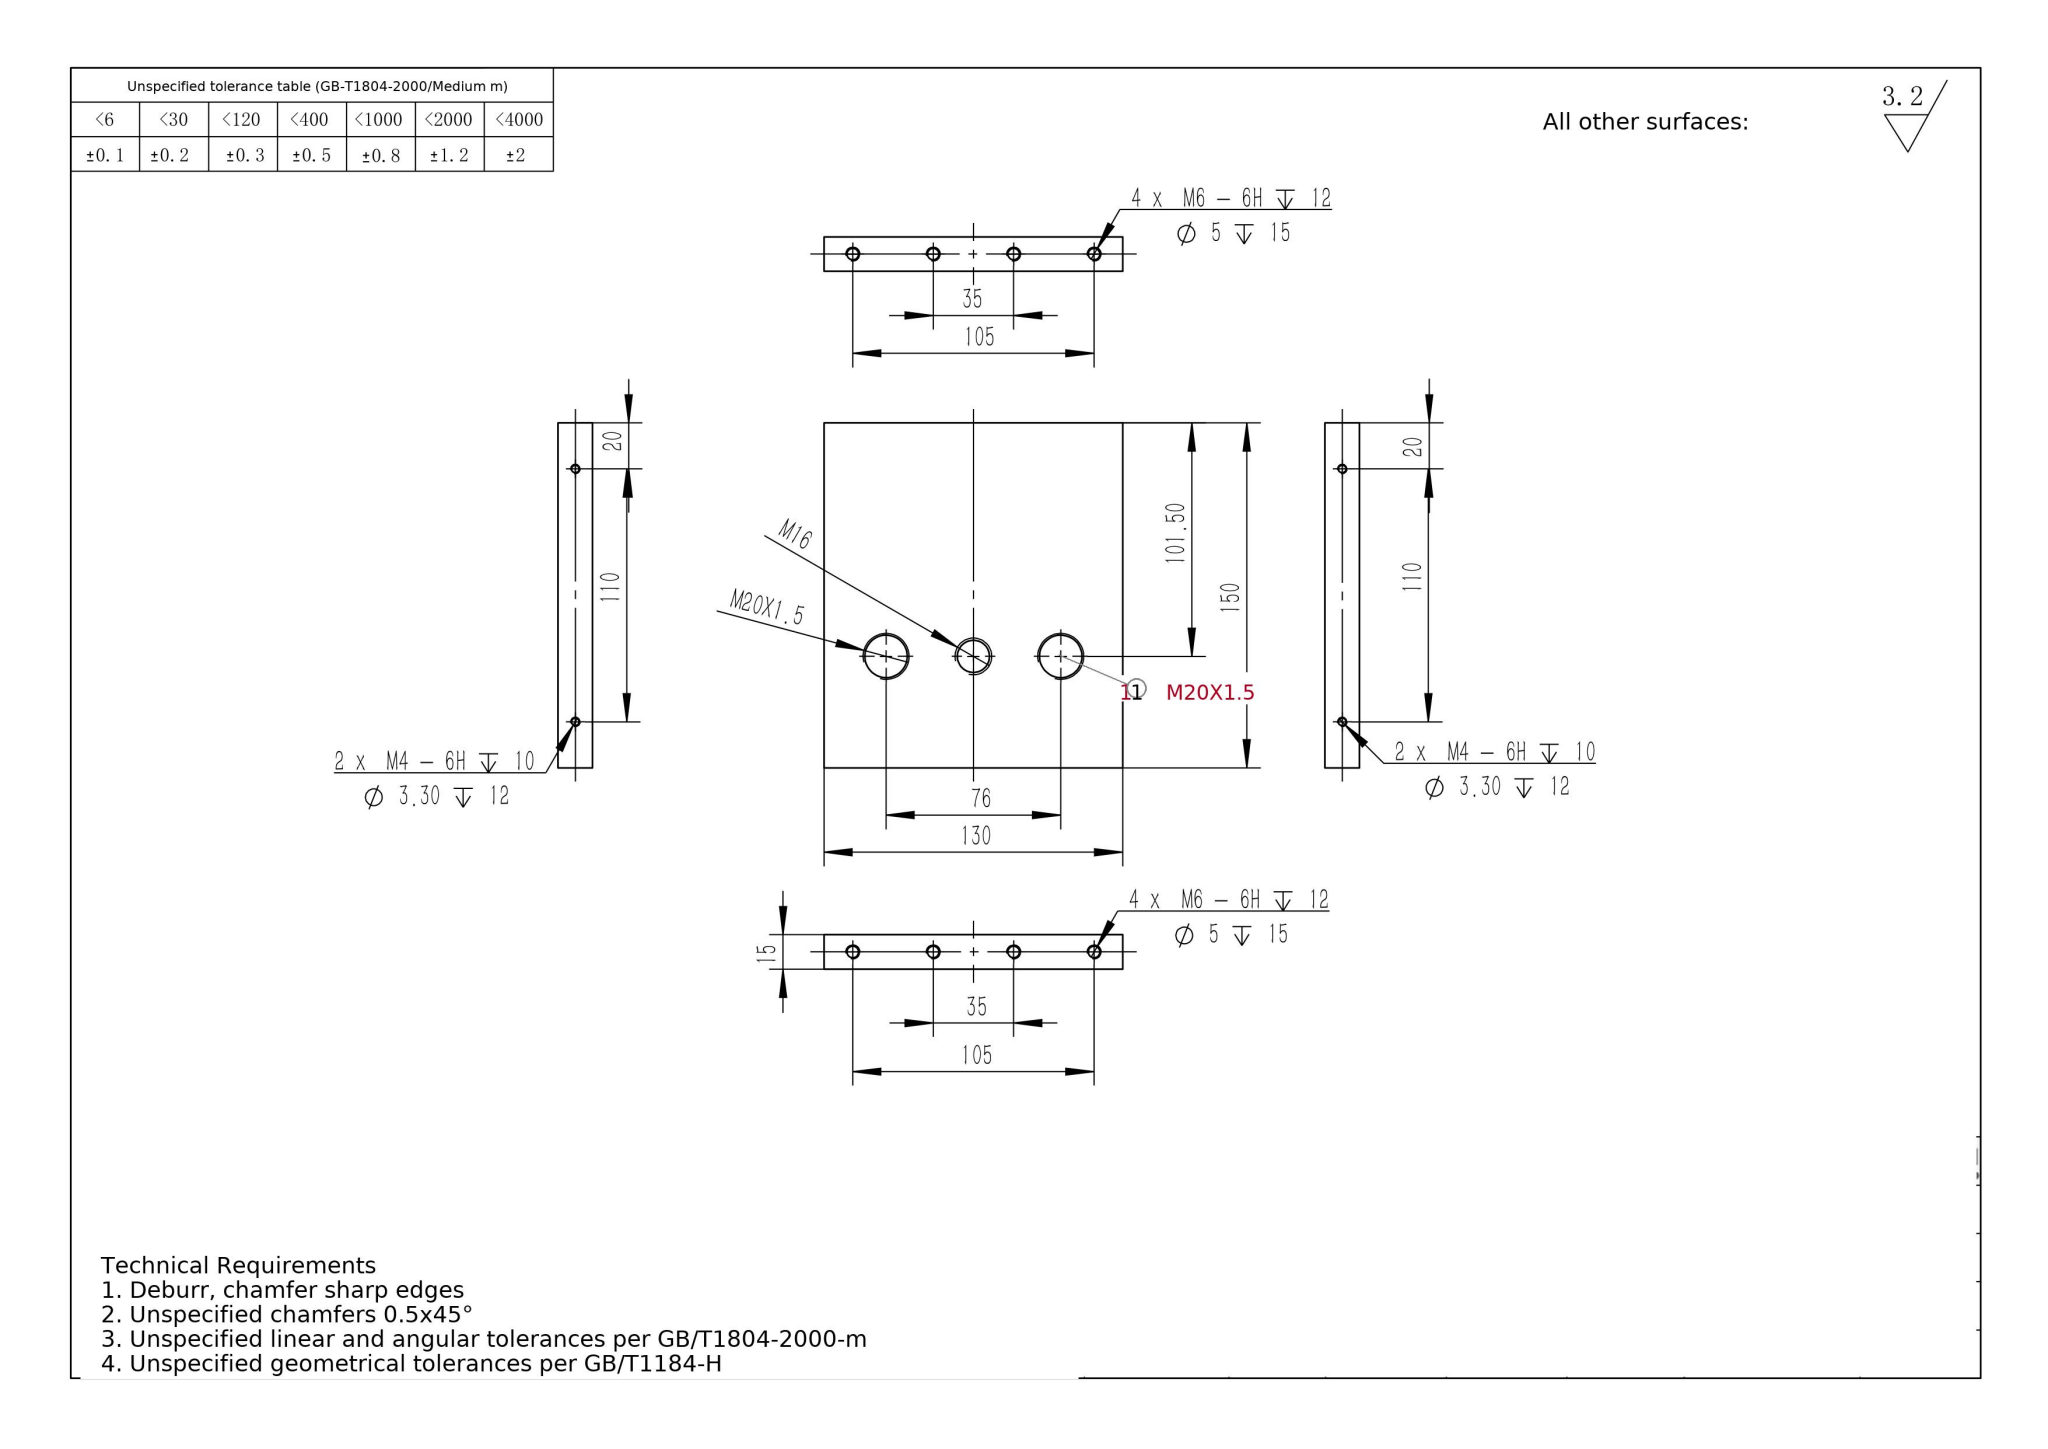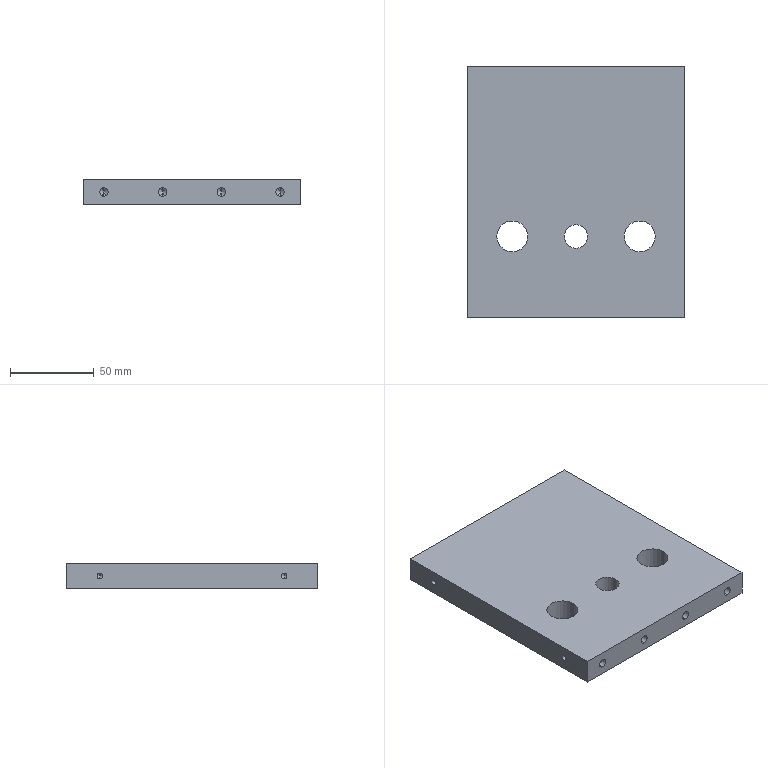Part | SolidWorks | mm | 1 solid | 60 faces | box 130 x 150 x 15 mm | volume 279270 mm3 | cylinder 30 | cone 24 | plane 6 | commonest cylinder face diameters 5 x16 3.3 x8 18.5 x4 14 x2
build123d program:
from build123d import *

# Parameters (mm, degrees)
SKETCH1_W                  = 130
SKETCH1_H                  = 150
BOSS_EXTRUDE1_DEPTH        = 15
M20X1_5_TAPPED_HOLE1_D     = 18.5
M20X1_5_TAPPED_HOLE1_DEPTH = 44.5
M20X1_5_TAPPED_HOLE1_TIP   = 5.558
M16_TAPPED_HOLE1_D         = 14
M16_TAPPED_HOLE1_DEPTH     = 38
M16_TAPPED_HOLE1_TIP       = 4.206
M6_TAPPED_HOLE1_AT_2_COUNT = 2
M6_TAPPED_HOLE1_AT_2_PITCH = 35
M6_TAPPED_HOLE1_AT_3_COUNT = 2
M6_TAPPED_HOLE1_AT_3_PITCH = 70
M6_TAPPED_HOLE1_AT_4_COUNT = 2
M6_TAPPED_HOLE1_AT_4_PITCH = 105
M4_TAPPED_HOLE1_AT_2_COUNT = 2
M4_TAPPED_HOLE1_AT_2_PITCH = 110


with BuildPart() as part:
    # Sketch1 → Boss-Extrude1 (new body)
    with BuildSketch(Plane.XY):
        with Locations((-65, -75)):
            Rectangle(SKETCH1_W, SKETCH1_H)
    extrude(amount=BOSS_EXTRUDE1_DEPTH)

    # M20x1.5 Tapped Hole1
    with Locations(Plane.XY.offset(15)):
        with Locations((-103, -101.5), (-27, -101.5)):
            Hole(M20X1_5_TAPPED_HOLE1_D / 2, depth=M20X1_5_TAPPED_HOLE1_DEPTH)
            with Locations((0, 0, -(M20X1_5_TAPPED_HOLE1_DEPTH + M20X1_5_TAPPED_HOLE1_TIP / 2))):  # 118° drill point
                Cone(0, M20X1_5_TAPPED_HOLE1_D / 2, M20X1_5_TAPPED_HOLE1_TIP, mode=Mode.SUBTRACT)

    # M16 Tapped Hole1
    with Locations(Plane.XY.offset(15)):
        with Locations((-65, -101.5)):
            Hole(M16_TAPPED_HOLE1_D / 2, depth=M16_TAPPED_HOLE1_DEPTH)
            with Locations((0, 0, -(M16_TAPPED_HOLE1_DEPTH + M16_TAPPED_HOLE1_TIP / 2))):  # 118° drill point
                Cone(0, M16_TAPPED_HOLE1_D / 2, M16_TAPPED_HOLE1_TIP, mode=Mode.SUBTRACT)

    # Sketch9 → M6 Tapped Hole1 (revolve, cut)
    with BuildSketch(Plane(origin=(-117.5, -150, 7.5), x_dir=(0, 0, -1), z_dir=(1, 0, 0))):
        Polygon((0, 0), (0, 16.502), (2.5, 15), (2.5, 0), align=None)
    m6_tapped_hole1 = revolve(axis=Axis((-117.5, -156.35, 7.5), (0, 1, 0)), mode=Mode.SUBTRACT)

    # M6 Tapped Hole1 at 2: M6 Tapped Hole1 ×2
    with Locations(*[(i * M6_TAPPED_HOLE1_AT_2_PITCH, 0, 0) for i in range(1, M6_TAPPED_HOLE1_AT_2_COUNT)]):
        add(m6_tapped_hole1, mode=Mode.SUBTRACT)

    # M6 Tapped Hole1 at 3: M6 Tapped Hole1 ×2
    with Locations(*[(i * M6_TAPPED_HOLE1_AT_3_PITCH, 0, 0) for i in range(1, M6_TAPPED_HOLE1_AT_3_COUNT)]):
        add(m6_tapped_hole1, mode=Mode.SUBTRACT)

    # M6 Tapped Hole1 at 4: M6 Tapped Hole1 ×2
    with Locations(*[(i * M6_TAPPED_HOLE1_AT_4_PITCH, 0, 0) for i in range(1, M6_TAPPED_HOLE1_AT_4_COUNT)]):
        add(m6_tapped_hole1, mode=Mode.SUBTRACT)

    # Mirror1: M6 Tapped Hole1 across plane
    add(m6_tapped_hole1.mirror(Plane.ZX.offset(-75)), mode=Mode.SUBTRACT)

    # Mirror1 copy 1 sketch → Mirror1 copy 1 (revolve, cut)
    with BuildSketch(Plane(origin=(-82.5, 0, 7.5), x_dir=(0, 0, -1), z_dir=(1, 0, 0))):
        Polygon((0, 0), (0, -16.502), (2.5, -15), (2.5, 0), align=None)
    revolve(axis=Axis((-82.5, 6.35, 7.5), (0, 1, 0)), mode=Mode.SUBTRACT)

    # Mirror1 copy 2 sketch → Mirror1 copy 2 (revolve, cut)
    with BuildSketch(Plane(origin=(-47.5, 0, 7.5), x_dir=(0, 0, -1), z_dir=(1, 0, 0))):
        Polygon((0, 0), (0, -16.502), (2.5, -15), (2.5, 0), align=None)
    revolve(axis=Axis((-47.5, 6.35, 7.5), (0, 1, 0)), mode=Mode.SUBTRACT)

    # Mirror1 copy 3 sketch → Mirror1 copy 3 (revolve, cut)
    with BuildSketch(Plane(origin=(-12.5, 0, 7.5), x_dir=(0, 0, -1), z_dir=(1, 0, 0))):
        Polygon((0, 0), (0, -16.502), (2.5, -15), (2.5, 0), align=None)
    revolve(axis=Axis((-12.5, 6.35, 7.5), (0, 1, 0)), mode=Mode.SUBTRACT)

    # Sketch11 → M4 Tapped Hole1 (revolve, cut)
    with BuildSketch(Plane(origin=(-130, -20, 7.5), x_dir=(0, 0, 1), z_dir=(0, 1, 0))):
        Polygon((0, 0), (0, 12.991), (1.65, 12), (1.65, 0), align=None)
    m4_tapped_hole1 = revolve(axis=Axis((-136.35, -20, 7.5), (1, 0, 0)), mode=Mode.SUBTRACT)

    # M4 Tapped Hole1 at 2: M4 Tapped Hole1 ×2
    with Locations(*[(0, -i * M4_TAPPED_HOLE1_AT_2_PITCH, 0) for i in range(1, M4_TAPPED_HOLE1_AT_2_COUNT)]):
        add(m4_tapped_hole1, mode=Mode.SUBTRACT)

    # Mirror2: M4 Tapped Hole1 across plane
    add(m4_tapped_hole1.mirror(Plane(origin=(-65, 0, 0), x_dir=(0, 0, 1), z_dir=(1, 0, 0))), mode=Mode.SUBTRACT)

    # Mirror2 copy 1 sketch → Mirror2 copy 1 (revolve, cut)
    with BuildSketch(Plane(origin=(0, -130, 7.5), x_dir=(0, 0, 1), z_dir=(0, 1, 0))):
        Polygon((0, 0), (0, -12.991), (1.65, -12), (1.65, 0), align=None)
    revolve(axis=Axis((6.35, -130, 7.5), (1, 0, 0)), mode=Mode.SUBTRACT)


solid = part.part